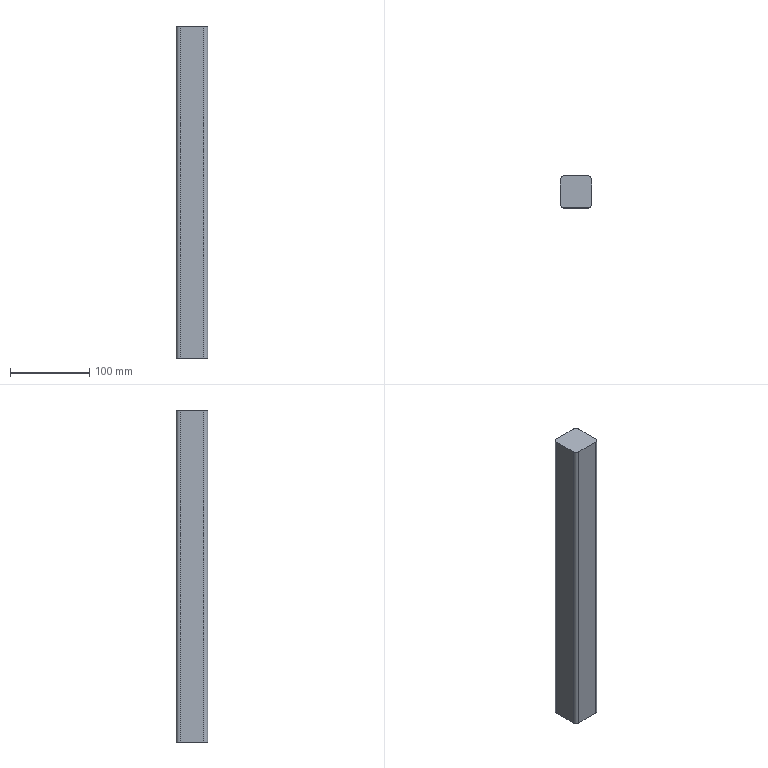Component | SolidWorks | Jig4040-420-1 | 1 solid | 10 faces | box 40 x 40 x 420 mm | volume 662987 mm3 | plane 6 | cylinder 4 | commonest cylinder face diameters 10 x4 | material Copper
build123d program:
from build123d import *

# Parameters (mm, degrees)
BOSS_EXTRUDE1_DEPTH = 420


with BuildPart() as part:
    # Sketch1 → Boss-Extrude1 (new body)
    with BuildSketch(Plane(origin=(0, 0, 0), x_dir=(1, 0, 0), z_dir=(0, 1, 0))):
        with BuildLine():
            Line((5, 0), (35, 0))
            ThreePointArc((35, 0), (38.536, 1.464), (40, 5))
            Line((40, 5), (40, 35))
            ThreePointArc((40, 35), (38.536, 38.536), (35, 40))
            Line((35, 40), (5, 40))
            ThreePointArc((5, 40), (1.464, 38.536), (0, 35))
            Line((0, 35), (0, 5))
            ThreePointArc((0, 5), (1.464, 1.464), (5, 0))
        make_face()
    extrude(amount=BOSS_EXTRUDE1_DEPTH)


solid = part.part

# Placed as in the assembly
solid = solid.moved(Location((-28.008, -107.909, 1370), (90, 0, 0)))
STEP:
#1=CARTESIAN_POINT('',(-0.9058,-2.674,53.937));
#2=VERTEX_POINT('',#1);
#3=CARTESIAN_POINT('',(-1.103,-2.87,53.937));
#4=VERTEX_POINT('',#3);
#5=CARTESIAN_POINT('',(-0.9058,-2.87,53.937));
#6=DIRECTION('',(0.,0.,1.));
#7=DIRECTION('',(0.,1.,0.));
#8=AXIS2_PLACEMENT_3D('',#5,#6,#7);
#9=CIRCLE('',#8,0.1969);
#10=EDGE_CURVE('',#2,#4,#9,.T.);
#11=ORIENTED_EDGE('',*,*,#10,.T.);
#12=CARTESIAN_POINT('',(-1.103,-2.87,70.472));
#13=VERTEX_POINT('',#12);
#14=CARTESIAN_POINT('',(-1.103,-2.87,70.472));
#15=DIRECTION('',(0.,-0.,-1.));
#16=VECTOR('',#15,39.37);
#17=LINE('',#14,#16);
#18=EDGE_CURVE('',#13,#4,#17,.T.);
#19=ORIENTED_EDGE('',*,*,#18,.F.);
#20=CARTESIAN_POINT('',(-0.9058,-2.674,70.472));
#21=VERTEX_POINT('',#20);
#22=CARTESIAN_POINT('',(-0.9058,-2.87,70.472));
#23=DIRECTION('',(0.,0.,1.));
#24=DIRECTION('',(0.,1.,0.));
#25=AXIS2_PLACEMENT_3D('',#22,#23,#24);
#26=CIRCLE('',#25,0.1969);
#27=EDGE_CURVE('',#21,#13,#26,.T.);
#28=ORIENTED_EDGE('',*,*,#27,.F.);
#29=CARTESIAN_POINT('',(-0.9058,-2.674,70.472));
#30=DIRECTION('',(0.,-0.,-1.));
#31=VECTOR('',#30,39.37);
#32=LINE('',#29,#31);
#33=EDGE_CURVE('',#21,#2,#32,.T.);
#34=ORIENTED_EDGE('',*,*,#33,.T.);
#35=EDGE_LOOP('',(#11,#19,#28,#34));
#36=FACE_OUTER_BOUND('',#35,.T.);
#37=CARTESIAN_POINT('',(-0.9058,-2.87,70.472));
#38=DIRECTION('',(0.,-0.,-1.));
#39=DIRECTION('',(0.,1.,0.));
#40=AXIS2_PLACEMENT_3D('',#37,#38,#39);
#41=CYLINDRICAL_SURFACE('',#40,0.1969);
#42=ADVANCED_FACE('',(#36),#41,.T.);
#43=CARTESIAN_POINT('',(-1.103,-4.052,53.937));
#44=VERTEX_POINT('',#43);
#45=CARTESIAN_POINT('',(-1.103,-4.052,53.937));
#46=DIRECTION('',(0.,-1.,0.));
#47=VECTOR('',#46,39.37);
#48=LINE('',#45,#47);
#49=EDGE_CURVE('',#4,#44,#48,.T.);
#50=ORIENTED_EDGE('',*,*,#49,.T.);
#51=CARTESIAN_POINT('',(-1.103,-4.052,70.472));
#52=VERTEX_POINT('',#51);
#53=CARTESIAN_POINT('',(-1.103,-4.052,70.472));
#54=DIRECTION('',(0.,-0.,-1.));
#55=VECTOR('',#54,39.37);
#56=LINE('',#53,#55);
#57=EDGE_CURVE('',#52,#44,#56,.T.);
#58=ORIENTED_EDGE('',*,*,#57,.F.);
#59=CARTESIAN_POINT('',(-1.103,-4.052,70.472));
#60=DIRECTION('',(0.,-1.,0.));
#61=VECTOR('',#60,39.37);
#62=LINE('',#59,#61);
#63=EDGE_CURVE('',#13,#52,#62,.T.);
#64=ORIENTED_EDGE('',*,*,#63,.F.);
#65=ORIENTED_EDGE('',*,*,#18,.T.);
#66=EDGE_LOOP('',(#50,#58,#64,#65));
#67=FACE_OUTER_BOUND('',#66,.T.);
#68=CARTESIAN_POINT('',(-1.103,-4.052,70.472));
#69=DIRECTION('',(1.,0.,0.));
#70=DIRECTION('',(0.,1.,-0.));
#71=AXIS2_PLACEMENT_3D('',#68,#69,#70);
#72=PLANE('',#71);
#73=ADVANCED_FACE('',(#67),#72,.F.);
#74=CARTESIAN_POINT('',(-0.9058,-4.248,53.937));
#75=VERTEX_POINT('',#74);
#76=CARTESIAN_POINT('',(-0.9058,-4.052,53.937));
#77=DIRECTION('',(0.,0.,1.));
#78=DIRECTION('',(0.,-1.,0.));
#79=AXIS2_PLACEMENT_3D('',#76,#77,#78);
#80=CIRCLE('',#79,0.1969);
#81=EDGE_CURVE('',#44,#75,#80,.T.);
#82=ORIENTED_EDGE('',*,*,#81,.T.);
#83=CARTESIAN_POINT('',(-0.9058,-4.248,70.472));
#84=VERTEX_POINT('',#83);
#85=CARTESIAN_POINT('',(-0.9058,-4.248,70.472));
#86=DIRECTION('',(0.,-0.,-1.));
#87=VECTOR('',#86,39.37);
#88=LINE('',#85,#87);
#89=EDGE_CURVE('',#84,#75,#88,.T.);
#90=ORIENTED_EDGE('',*,*,#89,.F.);
#91=CARTESIAN_POINT('',(-0.9058,-4.052,70.472));
#92=DIRECTION('',(0.,0.,1.));
#93=DIRECTION('',(0.,-1.,0.));
#94=AXIS2_PLACEMENT_3D('',#91,#92,#93);
#95=CIRCLE('',#94,0.1969);
#96=EDGE_CURVE('',#52,#84,#95,.T.);
#97=ORIENTED_EDGE('',*,*,#96,.F.);
#98=ORIENTED_EDGE('',*,*,#57,.T.);
#99=EDGE_LOOP('',(#82,#90,#97,#98));
#100=FACE_OUTER_BOUND('',#99,.T.);
#101=CARTESIAN_POINT('',(-0.9058,-4.052,70.472));
#102=DIRECTION('',(0.,-0.,-1.));
#103=DIRECTION('',(0.,1.,0.));
#104=AXIS2_PLACEMENT_3D('',#101,#102,#103);
#105=CYLINDRICAL_SURFACE('',#104,0.1969);
#106=ADVANCED_FACE('',(#100),#105,.T.);
#107=CARTESIAN_POINT('',(0.2753,-4.248,53.937));
#108=VERTEX_POINT('',#107);
#109=CARTESIAN_POINT('',(-0.9058,-4.248,53.937));
#110=DIRECTION('',(1.,0.,0.));
#111=VECTOR('',#110,39.37);
#112=LINE('',#109,#111);
#113=EDGE_CURVE('',#75,#108,#112,.T.);
#114=ORIENTED_EDGE('',*,*,#113,.T.);
#115=CARTESIAN_POINT('',(0.2753,-4.248,70.472));
#116=VERTEX_POINT('',#115);
#117=CARTESIAN_POINT('',(0.2753,-4.248,70.472));
#118=DIRECTION('',(0.,-0.,-1.));
#119=VECTOR('',#118,39.37);
#120=LINE('',#117,#119);
#121=EDGE_CURVE('',#116,#108,#120,.T.);
#122=ORIENTED_EDGE('',*,*,#121,.F.);
#123=CARTESIAN_POINT('',(-0.9058,-4.248,70.472));
#124=DIRECTION('',(1.,0.,0.));
#125=VECTOR('',#124,39.37);
#126=LINE('',#123,#125);
#127=EDGE_CURVE('',#84,#116,#126,.T.);
#128=ORIENTED_EDGE('',*,*,#127,.F.);
#129=ORIENTED_EDGE('',*,*,#89,.T.);
#130=EDGE_LOOP('',(#114,#122,#128,#129));
#131=FACE_OUTER_BOUND('',#130,.T.);
#132=CARTESIAN_POINT('',(-0.9058,-4.248,70.472));
#133=DIRECTION('',(0.,1.,-0.));
#134=DIRECTION('',(-1.,0.,0.));
#135=AXIS2_PLACEMENT_3D('',#132,#133,#134);
#136=PLANE('',#135);
#137=ADVANCED_FACE('',(#131),#136,.F.);
#138=CARTESIAN_POINT('',(0.4721,-4.052,53.937));
#139=VERTEX_POINT('',#138);
#140=CARTESIAN_POINT('',(0.2753,-4.052,53.937));
#141=DIRECTION('',(0.,0.,1.));
#142=DIRECTION('',(0.,-1.,0.));
#143=AXIS2_PLACEMENT_3D('',#140,#141,#142);
#144=CIRCLE('',#143,0.1969);
#145=EDGE_CURVE('',#108,#139,#144,.T.);
#146=ORIENTED_EDGE('',*,*,#145,.T.);
#147=CARTESIAN_POINT('',(0.4721,-4.052,70.472));
#148=VERTEX_POINT('',#147);
#149=CARTESIAN_POINT('',(0.4721,-4.052,70.472));
#150=DIRECTION('',(0.,-0.,-1.));
#151=VECTOR('',#150,39.37);
#152=LINE('',#149,#151);
#153=EDGE_CURVE('',#148,#139,#152,.T.);
#154=ORIENTED_EDGE('',*,*,#153,.F.);
#155=CARTESIAN_POINT('',(0.2753,-4.052,70.472));
#156=DIRECTION('',(0.,0.,1.));
#157=DIRECTION('',(0.,-1.,0.));
#158=AXIS2_PLACEMENT_3D('',#155,#156,#157);
#159=CIRCLE('',#158,0.1969);
#160=EDGE_CURVE('',#116,#148,#159,.T.);
#161=ORIENTED_EDGE('',*,*,#160,.F.);
#162=ORIENTED_EDGE('',*,*,#121,.T.);
#163=EDGE_LOOP('',(#146,#154,#161,#162));
#164=FACE_OUTER_BOUND('',#163,.T.);
#165=CARTESIAN_POINT('',(0.2753,-4.052,70.472));
#166=DIRECTION('',(0.,-0.,-1.));
#167=DIRECTION('',(0.,1.,0.));
#168=AXIS2_PLACEMENT_3D('',#165,#166,#167);
#169=CYLINDRICAL_SURFACE('',#168,0.1969);
#170=ADVANCED_FACE('',(#164),#169,.T.);
#171=CARTESIAN_POINT('',(0.4721,-2.87,53.937));
#172=VERTEX_POINT('',#171);
#173=CARTESIAN_POINT('',(0.4721,-4.052,53.937));
#174=DIRECTION('',(0.,1.,-0.));
#175=VECTOR('',#174,39.37);
#176=LINE('',#173,#175);
#177=EDGE_CURVE('',#139,#172,#176,.T.);
#178=ORIENTED_EDGE('',*,*,#177,.T.);
#179=CARTESIAN_POINT('',(0.4721,-2.87,70.472));
#180=VERTEX_POINT('',#179);
#181=CARTESIAN_POINT('',(0.4721,-2.87,70.472));
#182=DIRECTION('',(0.,-0.,-1.));
#183=VECTOR('',#182,39.37);
#184=LINE('',#181,#183);
#185=EDGE_CURVE('',#180,#172,#184,.T.);
#186=ORIENTED_EDGE('',*,*,#185,.F.);
#187=CARTESIAN_POINT('',(0.4721,-4.052,70.472));
#188=DIRECTION('',(0.,1.,-0.));
#189=VECTOR('',#188,39.37);
#190=LINE('',#187,#189);
#191=EDGE_CURVE('',#148,#180,#190,.T.);
#192=ORIENTED_EDGE('',*,*,#191,.F.);
#193=ORIENTED_EDGE('',*,*,#153,.T.);
#194=EDGE_LOOP('',(#178,#186,#192,#193));
#195=FACE_OUTER_BOUND('',#194,.T.);
#196=CARTESIAN_POINT('',(0.4721,-4.052,70.472));
#197=DIRECTION('',(-1.,0.,0.));
#198=DIRECTION('',(0.,-1.,0.));
#199=AXIS2_PLACEMENT_3D('',#196,#197,#198);
#200=PLANE('',#199);
#201=ADVANCED_FACE('',(#195),#200,.F.);
#202=CARTESIAN_POINT('',(0.2753,-2.674,53.937));
#203=VERTEX_POINT('',#202);
#204=CARTESIAN_POINT('',(0.2753,-2.87,53.937));
#205=DIRECTION('',(0.,0.,1.));
#206=DIRECTION('',(0.,-1.,0.));
#207=AXIS2_PLACEMENT_3D('',#204,#205,#206);
#208=CIRCLE('',#207,0.1969);
#209=EDGE_CURVE('',#172,#203,#208,.T.);
#210=ORIENTED_EDGE('',*,*,#209,.T.);
#211=CARTESIAN_POINT('',(0.2753,-2.674,70.472));
#212=VERTEX_POINT('',#211);
#213=CARTESIAN_POINT('',(0.2753,-2.674,70.472));
#214=DIRECTION('',(0.,-0.,-1.));
#215=VECTOR('',#214,39.37);
#216=LINE('',#213,#215);
#217=EDGE_CURVE('',#212,#203,#216,.T.);
#218=ORIENTED_EDGE('',*,*,#217,.F.);
#219=CARTESIAN_POINT('',(0.2753,-2.87,70.472));
#220=DIRECTION('',(0.,0.,1.));
#221=DIRECTION('',(0.,-1.,0.));
#222=AXIS2_PLACEMENT_3D('',#219,#220,#221);
#223=CIRCLE('',#222,0.1969);
#224=EDGE_CURVE('',#180,#212,#223,.T.);
#225=ORIENTED_EDGE('',*,*,#224,.F.);
#226=ORIENTED_EDGE('',*,*,#185,.T.);
#227=EDGE_LOOP('',(#210,#218,#225,#226));
#228=FACE_OUTER_BOUND('',#227,.T.);
#229=CARTESIAN_POINT('',(0.2753,-2.87,70.472));
#230=DIRECTION('',(0.,-0.,-1.));
#231=DIRECTION('',(0.,1.,0.));
#232=AXIS2_PLACEMENT_3D('',#229,#230,#231);
#233=CYLINDRICAL_SURFACE('',#232,0.1969);
#234=ADVANCED_FACE('',(#228),#233,.T.);
#235=CARTESIAN_POINT('',(-0.9058,-2.674,53.937));
#236=DIRECTION('',(-1.,0.,0.));
#237=VECTOR('',#236,39.37);
#238=LINE('',#235,#237);
#239=EDGE_CURVE('',#203,#2,#238,.T.);
#240=ORIENTED_EDGE('',*,*,#239,.T.);
#241=ORIENTED_EDGE('',*,*,#33,.F.);
#242=CARTESIAN_POINT('',(-0.9058,-2.674,70.472));
#243=DIRECTION('',(-1.,0.,0.));
#244=VECTOR('',#243,39.37);
#245=LINE('',#242,#244);
#246=EDGE_CURVE('',#212,#21,#245,.T.);
#247=ORIENTED_EDGE('',*,*,#246,.F.);
#248=ORIENTED_EDGE('',*,*,#217,.T.);
#249=EDGE_LOOP('',(#240,#241,#247,#248));
#250=FACE_OUTER_BOUND('',#249,.T.);
#251=CARTESIAN_POINT('',(-0.9058,-2.674,70.472));
#252=DIRECTION('',(0.,-1.,0.));
#253=DIRECTION('',(1.,0.,0.));
#254=AXIS2_PLACEMENT_3D('',#251,#252,#253);
#255=PLANE('',#254);
#256=ADVANCED_FACE('',(#250),#255,.F.);
#257=ORIENTED_EDGE('',*,*,#27,.T.);
#258=ORIENTED_EDGE('',*,*,#63,.T.);
#259=ORIENTED_EDGE('',*,*,#96,.T.);
#260=ORIENTED_EDGE('',*,*,#127,.T.);
#261=ORIENTED_EDGE('',*,*,#160,.T.);
#262=ORIENTED_EDGE('',*,*,#191,.T.);
#263=ORIENTED_EDGE('',*,*,#224,.T.);
#264=ORIENTED_EDGE('',*,*,#246,.T.);
#265=EDGE_LOOP('',(#257,#258,#259,#260,#261,#262,#263,#264));
#266=FACE_OUTER_BOUND('',#265,.T.);
#267=CARTESIAN_POINT('',(-0.9058,-2.87,70.472));
#268=DIRECTION('',(0.,-0.,-1.));
#269=DIRECTION('',(0.,1.,-0.));
#270=AXIS2_PLACEMENT_3D('',#267,#268,#269);
#271=PLANE('',#270);
#272=ADVANCED_FACE('',(#266),#271,.F.);
#273=ORIENTED_EDGE('',*,*,#10,.F.);
#274=ORIENTED_EDGE('',*,*,#239,.F.);
#275=ORIENTED_EDGE('',*,*,#209,.F.);
#276=ORIENTED_EDGE('',*,*,#177,.F.);
#277=ORIENTED_EDGE('',*,*,#145,.F.);
#278=ORIENTED_EDGE('',*,*,#113,.F.);
#279=ORIENTED_EDGE('',*,*,#81,.F.);
#280=ORIENTED_EDGE('',*,*,#49,.F.);
#281=EDGE_LOOP('',(#273,#274,#275,#276,#277,#278,#279,#280));
#282=FACE_OUTER_BOUND('',#281,.T.);
#283=CARTESIAN_POINT('',(-0.9058,-2.87,53.937));
#284=DIRECTION('',(0.,-0.,-1.));
#285=DIRECTION('',(0.,1.,-0.));
#286=AXIS2_PLACEMENT_3D('',#283,#284,#285);
#287=PLANE('',#286);
#288=ADVANCED_FACE('',(#282),#287,.T.);
#289=CLOSED_SHELL('',(#42,#73,#106,#137,#170,#201,#234,#256,#272,#288));
#290=MANIFOLD_SOLID_BREP('',#289);
#291=CARTESIAN_POINT('',(0.,0.,0.));
#292=DIRECTION('',(0.,0.,1.));
#293=DIRECTION('',(1.,0.,0.));
#294=AXIS2_PLACEMENT_3D('',#291,#292,#293);
#295=(LENGTH_UNIT()NAMED_UNIT(*)SI_UNIT($,.METRE.));
#296=LENGTH_MEASURE_WITH_UNIT(LENGTH_MEASURE(0.0254),#295);
#297=DIMENSIONAL_EXPONENTS(1.,0.,0.,0.,0.,0.,0.);
#298=(CONVERSION_BASED_UNIT('',#296)LENGTH_UNIT()NAMED_UNIT(#297));
#299=UNCERTAINTY_MEASURE_WITH_UNIT(LENGTH_MEASURE(0.00001),#298,'','');
#300=(NAMED_UNIT(*)PLANE_ANGLE_UNIT()SI_UNIT($,.RADIAN.));
#301=(NAMED_UNIT(*)SI_UNIT($,.STERADIAN.)SOLID_ANGLE_UNIT());
#302=(GEOMETRIC_REPRESENTATION_CONTEXT(3)GLOBAL_UNCERTAINTY_ASSIGNED_CONTEXT((#299))GLOBAL_UNIT_ASSIGNED_CONTEXT((#298,#300,#301))REPRESENTATION_CONTEXT('',''));
#303=ADVANCED_BREP_SHAPE_REPRESENTATION('',(#290,#294),#302);
#304=COLOUR_RGB('',0.7922,0.8196,0.9333);
#305=FILL_AREA_STYLE_COLOUR('',#304);
#306=FILL_AREA_STYLE('',(#305));
#307=SURFACE_STYLE_FILL_AREA(#306);
#308=SURFACE_SIDE_STYLE('',(#307));
#309=SURFACE_STYLE_USAGE(.BOTH.,#308);
#310=PRESENTATION_STYLE_ASSIGNMENT((#309));
#311=STYLED_ITEM('',(#310),#290);
#312=(LENGTH_UNIT()NAMED_UNIT(*)SI_UNIT($,.METRE.));
#313=LENGTH_MEASURE_WITH_UNIT(LENGTH_MEASURE(0.0254),#312);
#314=DIMENSIONAL_EXPONENTS(1.,0.,0.,0.,0.,0.,0.);
#315=(CONVERSION_BASED_UNIT('',#313)LENGTH_UNIT()NAMED_UNIT(#314));
#316=UNCERTAINTY_MEASURE_WITH_UNIT(LENGTH_MEASURE(0.00001),#315,'','');
#317=(NAMED_UNIT(*)PLANE_ANGLE_UNIT()SI_UNIT($,.RADIAN.));
#318=(NAMED_UNIT(*)SI_UNIT($,.STERADIAN.)SOLID_ANGLE_UNIT());
#319=(GEOMETRIC_REPRESENTATION_CONTEXT(3)GLOBAL_UNCERTAINTY_ASSIGNED_CONTEXT((#316))GLOBAL_UNIT_ASSIGNED_CONTEXT((#315,#317,#318))REPRESENTATION_CONTEXT('',''));
#320=MECHANICAL_DESIGN_GEOMETRIC_PRESENTATION_REPRESENTATION('',(#311),#319);
#321=PRESENTATION_LAYER_ASSIGNMENT('','',(#311));